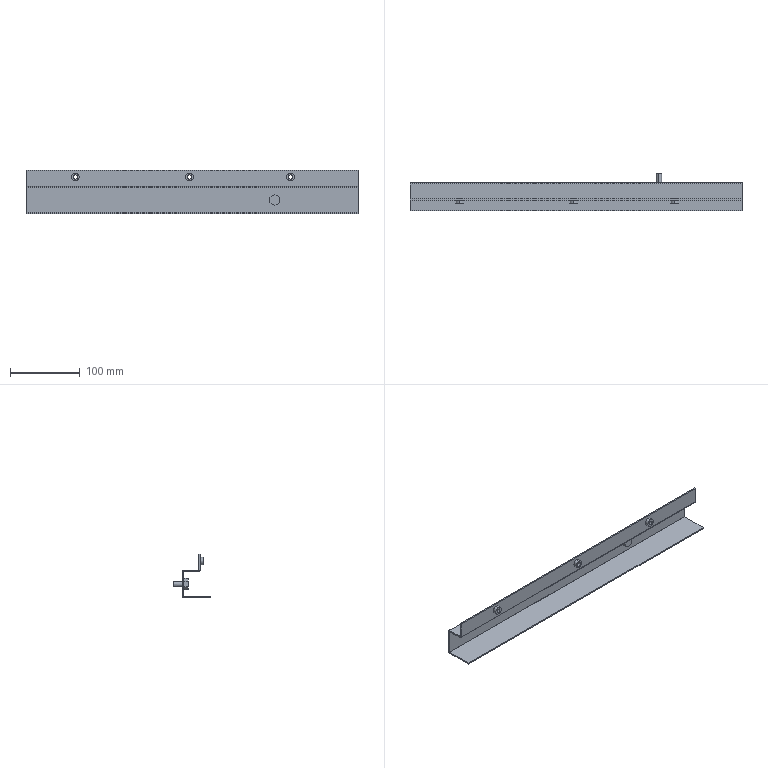Component | SolidWorks | CabinetWelding-1_ShelfSupportBeamLeft-1 | 1 solid | 63 faces | volume 108416 mm3 | plane 35 | cylinder 28 | commonest cylinder face diameters 8 x8 6 x6 11 x6 0.2 x3 3.8 x3 7.99 x2